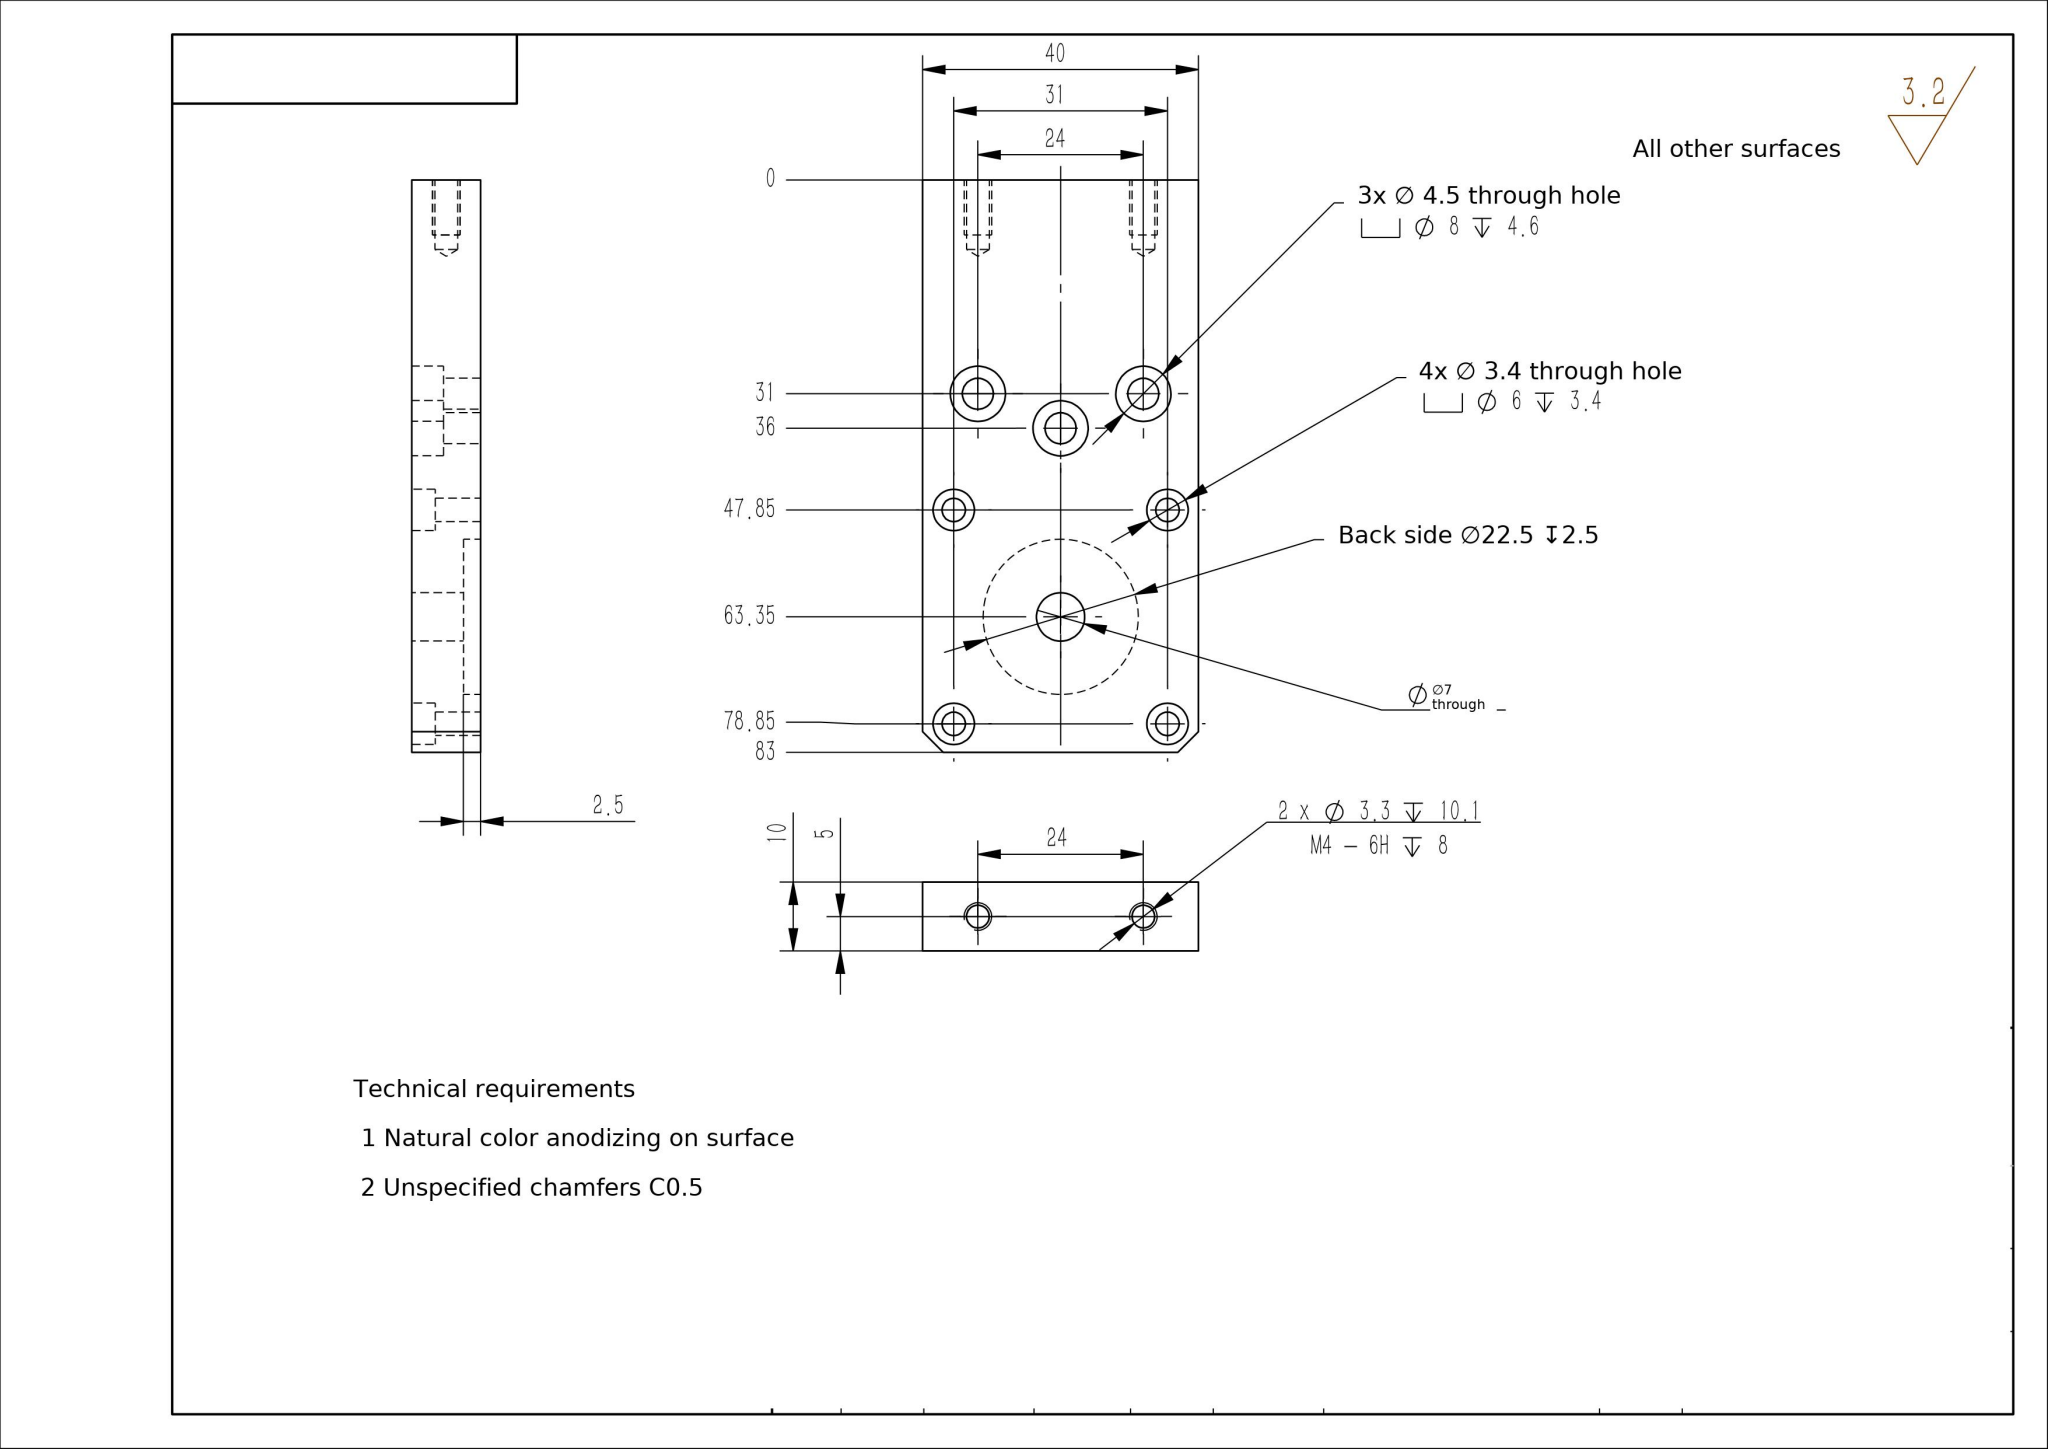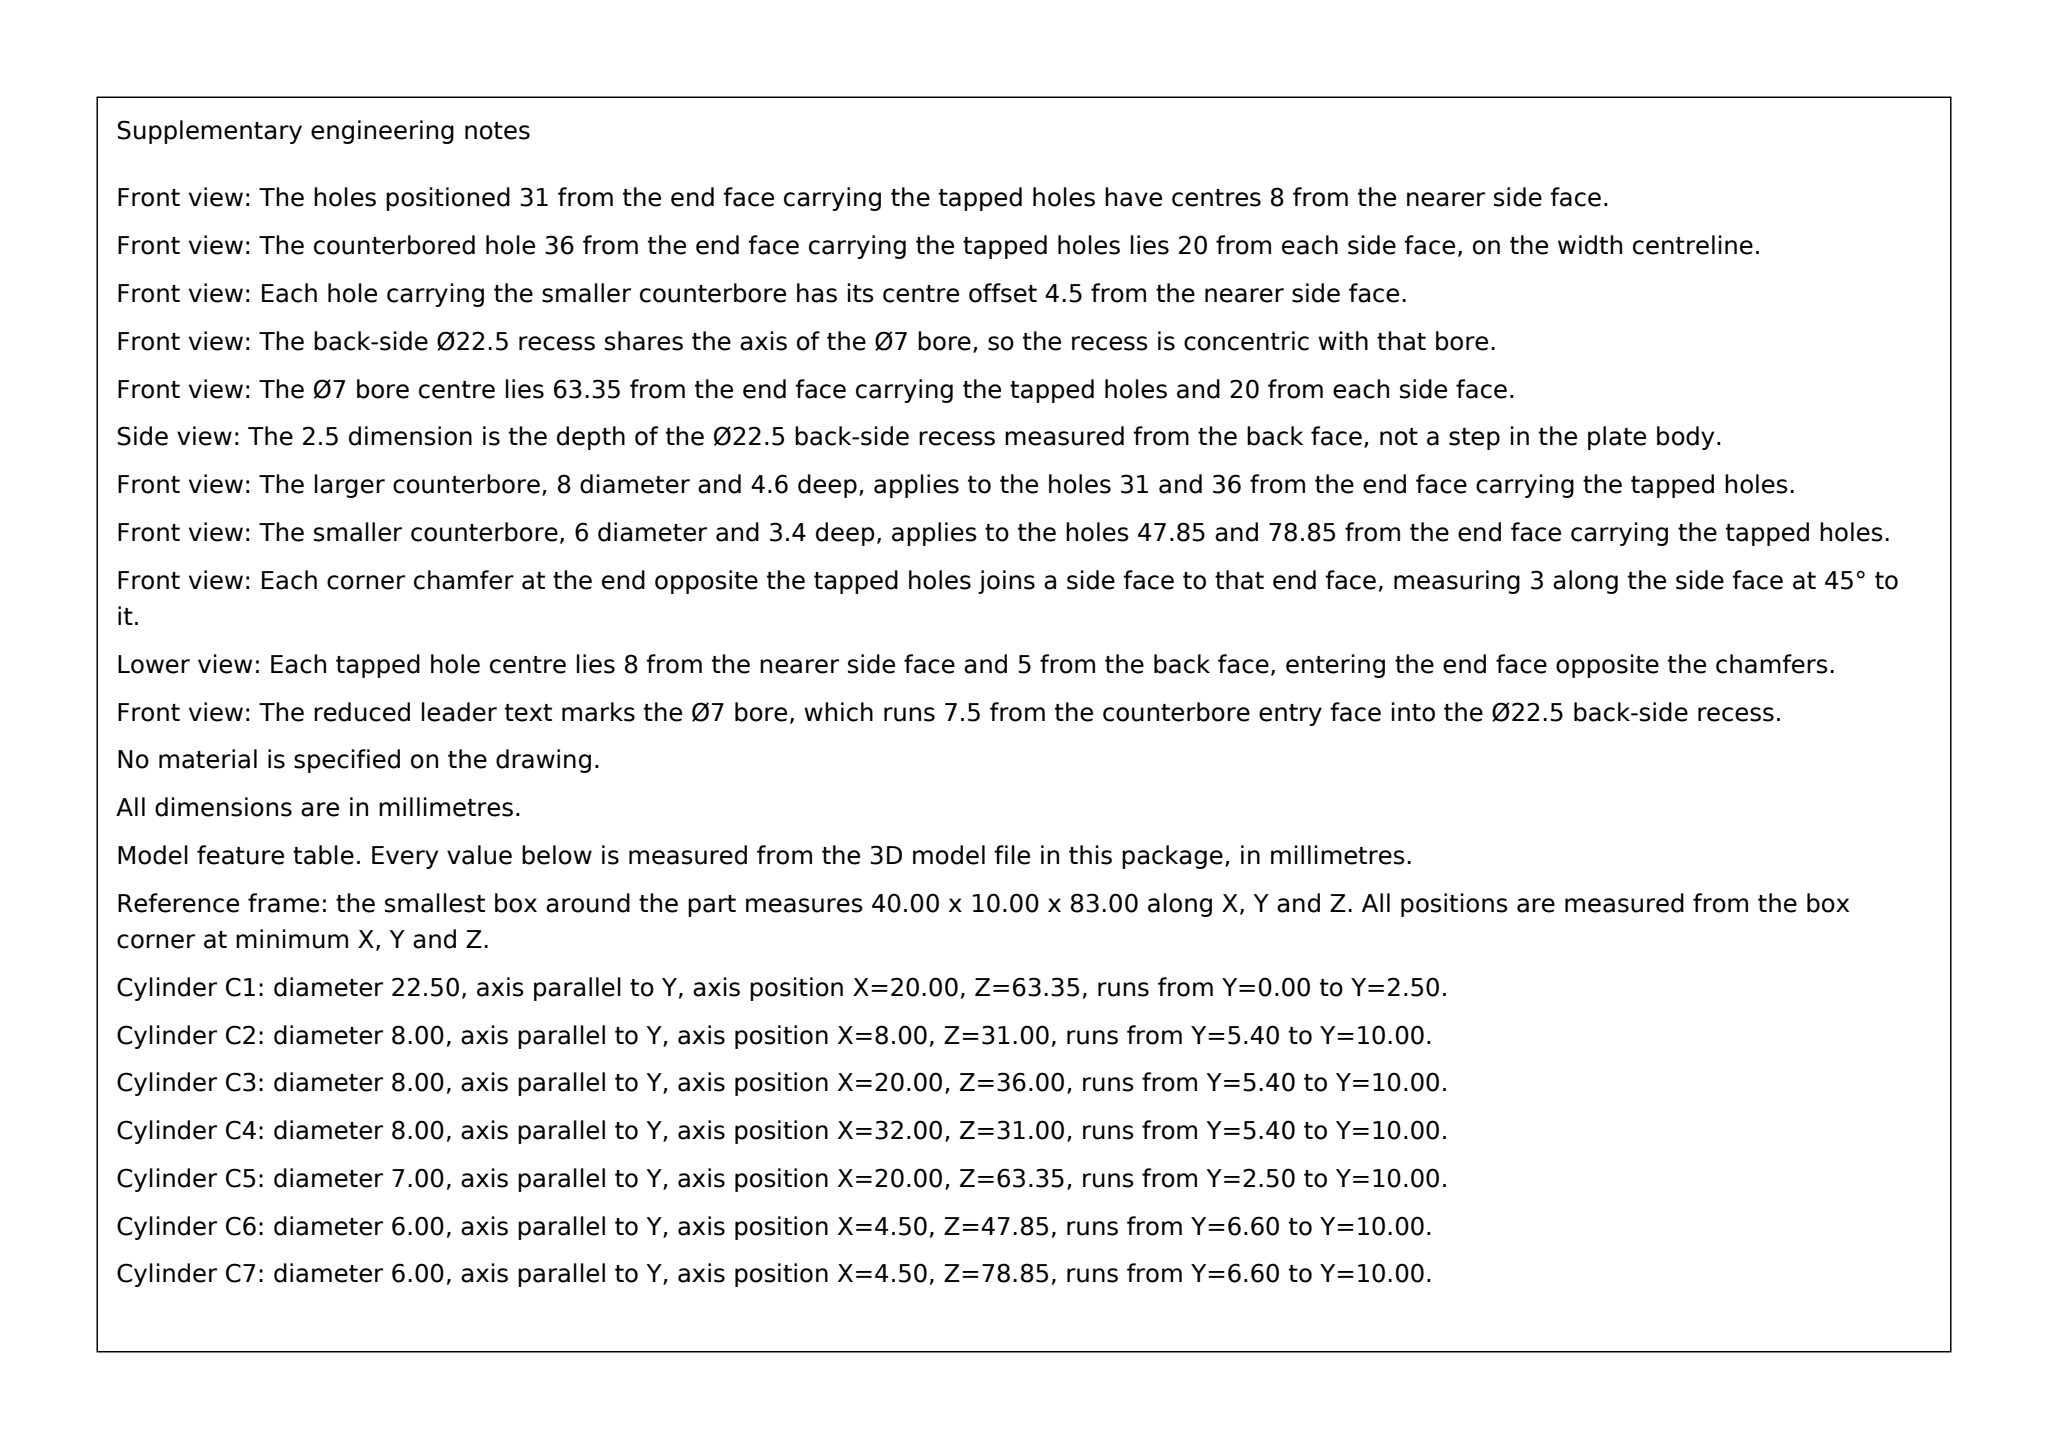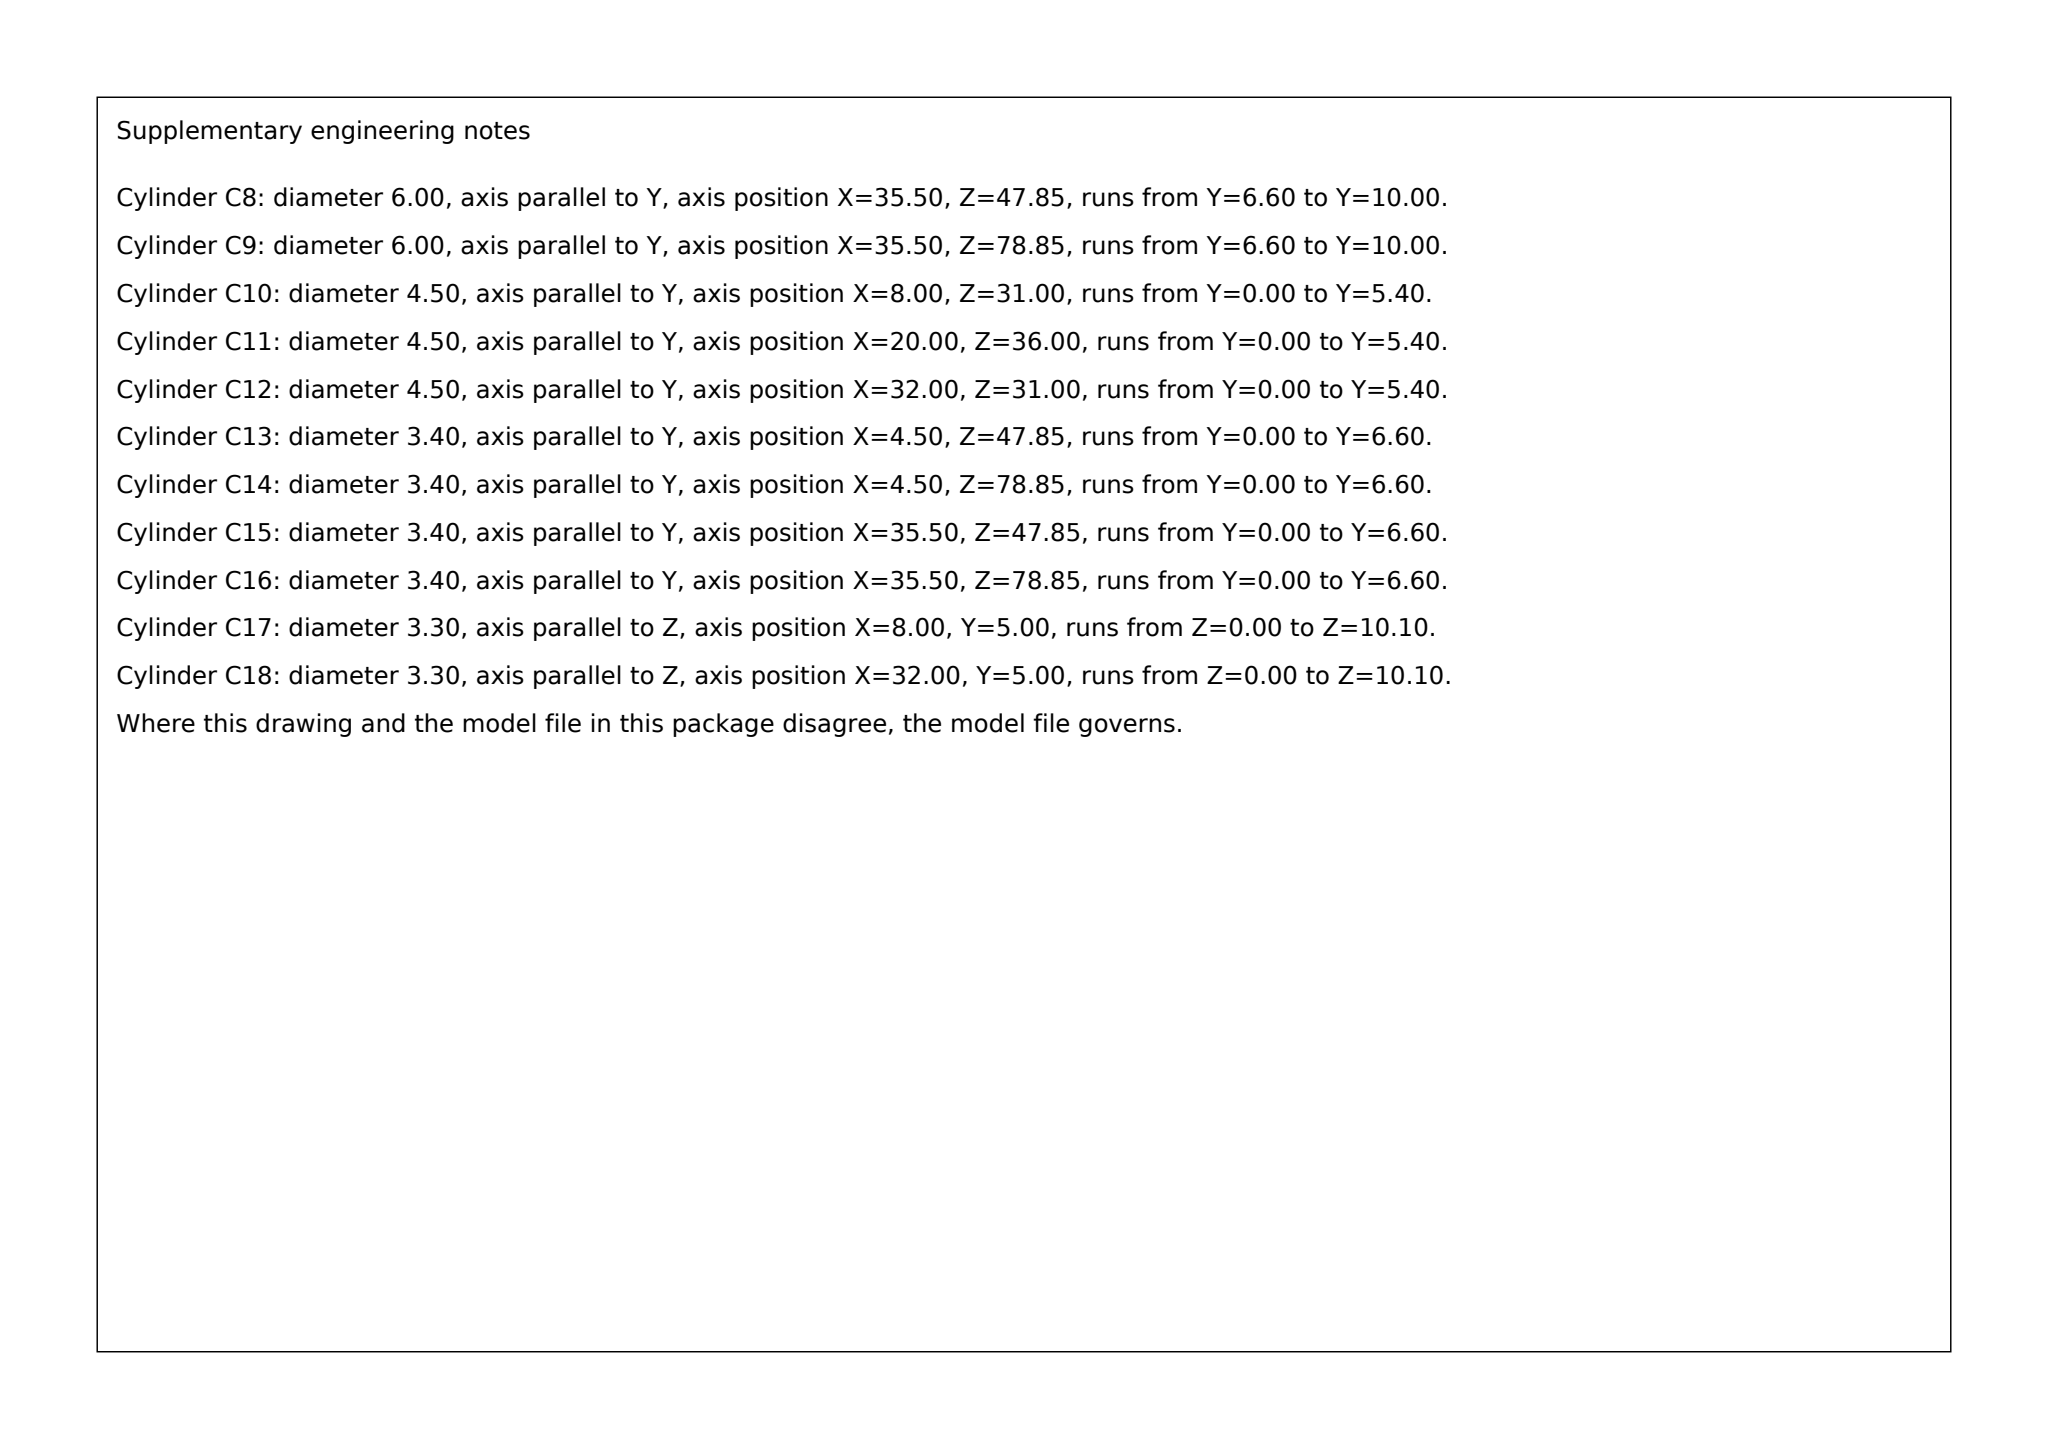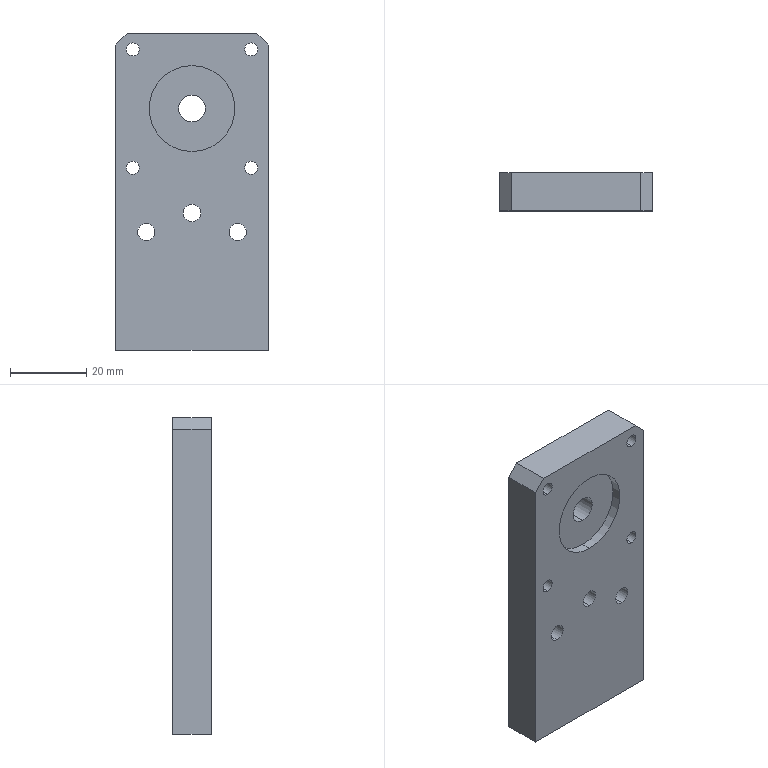Part | SolidWorks | mm | 1 solid | 56 faces | box 40 x 10 x 83 mm | volume 30073 mm3 | cylinder 36 | plane 16 | cone 4 | commonest cylinder face diameters 6 x8 3.4 x8 8 x6 4.5 x6 3.3 x4 7 x2 22.5 x2
Drawing notes:
Ø7 THRU ON VERT CL, 63.35 FROM TOP EDGE (0 DATUM) | from the solid: cylinder dia 7.0, axis y, pos x=20.0 (CL of 40 wide), z=63.35, length 7.5 = full 10 thk less Ø22.5 x 2.5 back c'bore
build123d program:
from build123d import *

# Parameters (mm, degrees)
SKETCH1_W                                        = 40
SKETCH1_H                                        = 63
BOSS_EXTRUDE1_DEPTH                              = 10
SKETCH3_R                                        = 11.25
CUT_EXTRUDE1_DEPTH                               = 2.5
SKETCH4_R                                        = 3.5
CUT_EXTRUDE2_DEPTH                               = 39.059
HOLE_SIZE_ACCORDING_TO_TYPE_2_OF_HEX_D           = 3.4
HOLE_SIZE_ACCORDING_TO_TYPE_2_OF_HEX_CBORE_D     = 6
HOLE_SIZE_ACCORDING_TO_TYPE_2_OF_HEX_CBORE_DEPTH = 3.4
CHAMFER1_SIZE                                    = 3
HOLE_SIZE_ACCORDING_TO_TYPE_3_OF_HEX_D           = 4.5
HOLE_SIZE_ACCORDING_TO_TYPE_3_OF_HEX_CBORE_D     = 8
HOLE_SIZE_ACCORDING_TO_TYPE_3_OF_HEX_CBORE_DEPTH = 4.6
SKETCH13_W                                       = 40
SKETCH13_H                                       = 20
BOSS_EXTRUDE2_DEPTH                              = 10
M4_TAPPED_HOLE1_D                                = 3.3
M4_TAPPED_HOLE1_DEPTH                            = 10.1
M4_TAPPED_HOLE1_TIP                              = 0.9914


with BuildPart() as part:
    # Sketch1 → Boss-Extrude1 (new body)
    with BuildSketch(Plane(origin=(0, 0, 0), x_dir=(1, 0, 0), z_dir=(0, 1, 0))):
        Rectangle(SKETCH1_W, SKETCH1_H)
    extrude(amount=BOSS_EXTRUDE1_DEPTH)

    # Sketch3 → Cut-Extrude1 (cut)
    with BuildSketch(Plane.XZ):
        with Locations(Location((0, 11.85, 0), (0, 0, 270))):
            Circle(SKETCH3_R)
    extrude(amount=-CUT_EXTRUDE1_DEPTH, mode=Mode.SUBTRACT)

    # Sketch4 → Cut-Extrude2 (cut, through all)
    with BuildSketch(Plane.XZ.offset(-2.5)):
        with Locations(Location((0, 11.85, 0), (0, 0, 270))):
            Circle(SKETCH4_R)
    extrude(amount=-CUT_EXTRUDE2_DEPTH, mode=Mode.SUBTRACT)

    # Hole Size _ according to_ type 2 of hex (through all)
    with Locations(Plane(origin=(0, 10, 0), x_dir=(1, 0, 0), z_dir=(0, 1, 0))):
        with Locations((-15.5, 3.65), (15.5, 3.65), (15.5, -27.35), (-15.5, -27.35)):
            CounterBoreHole(HOLE_SIZE_ACCORDING_TO_TYPE_2_OF_HEX_D / 2, HOLE_SIZE_ACCORDING_TO_TYPE_2_OF_HEX_CBORE_D / 2, HOLE_SIZE_ACCORDING_TO_TYPE_2_OF_HEX_CBORE_DEPTH)

    # Chamfer1
    chamfer1_edges = [part.edges().sort_by_distance(p)[0] for p in [
        (20, 5, 31.5),
        (-20, 5, 31.5),
    ]]
    chamfer(chamfer1_edges, length=CHAMFER1_SIZE)

    # Hole Size _ according to_ type 3 of hex (through all)
    with Locations(Plane(origin=(0, 10, 0), x_dir=(1, 0, 0), z_dir=(0, 1, 0))):
        with Locations((-12, 20.5), (12, 20.5), (0, 15.5)):
            CounterBoreHole(HOLE_SIZE_ACCORDING_TO_TYPE_3_OF_HEX_D / 2, HOLE_SIZE_ACCORDING_TO_TYPE_3_OF_HEX_CBORE_D / 2, HOLE_SIZE_ACCORDING_TO_TYPE_3_OF_HEX_CBORE_DEPTH)

    # Sketch13 → Boss-Extrude2 (add)
    with BuildSketch(Plane.XZ):
        with Locations((0, -41.5)):
            Rectangle(SKETCH13_W, SKETCH13_H)
    extrude(amount=-BOSS_EXTRUDE2_DEPTH)

    # M4 Tapped Hole1
    with Locations(Plane(origin=(0, 0, -51.5), x_dir=(-1, 0, 0), z_dir=(0, 0, -1))):
        with Locations((12, 5), (-12, 5)):
            Hole(M4_TAPPED_HOLE1_D / 2, depth=M4_TAPPED_HOLE1_DEPTH)
            with Locations((0, 0, -(M4_TAPPED_HOLE1_DEPTH + M4_TAPPED_HOLE1_TIP / 2))):  # 118° drill point
                Cone(0, M4_TAPPED_HOLE1_D / 2, M4_TAPPED_HOLE1_TIP, mode=Mode.SUBTRACT)


solid = part.part